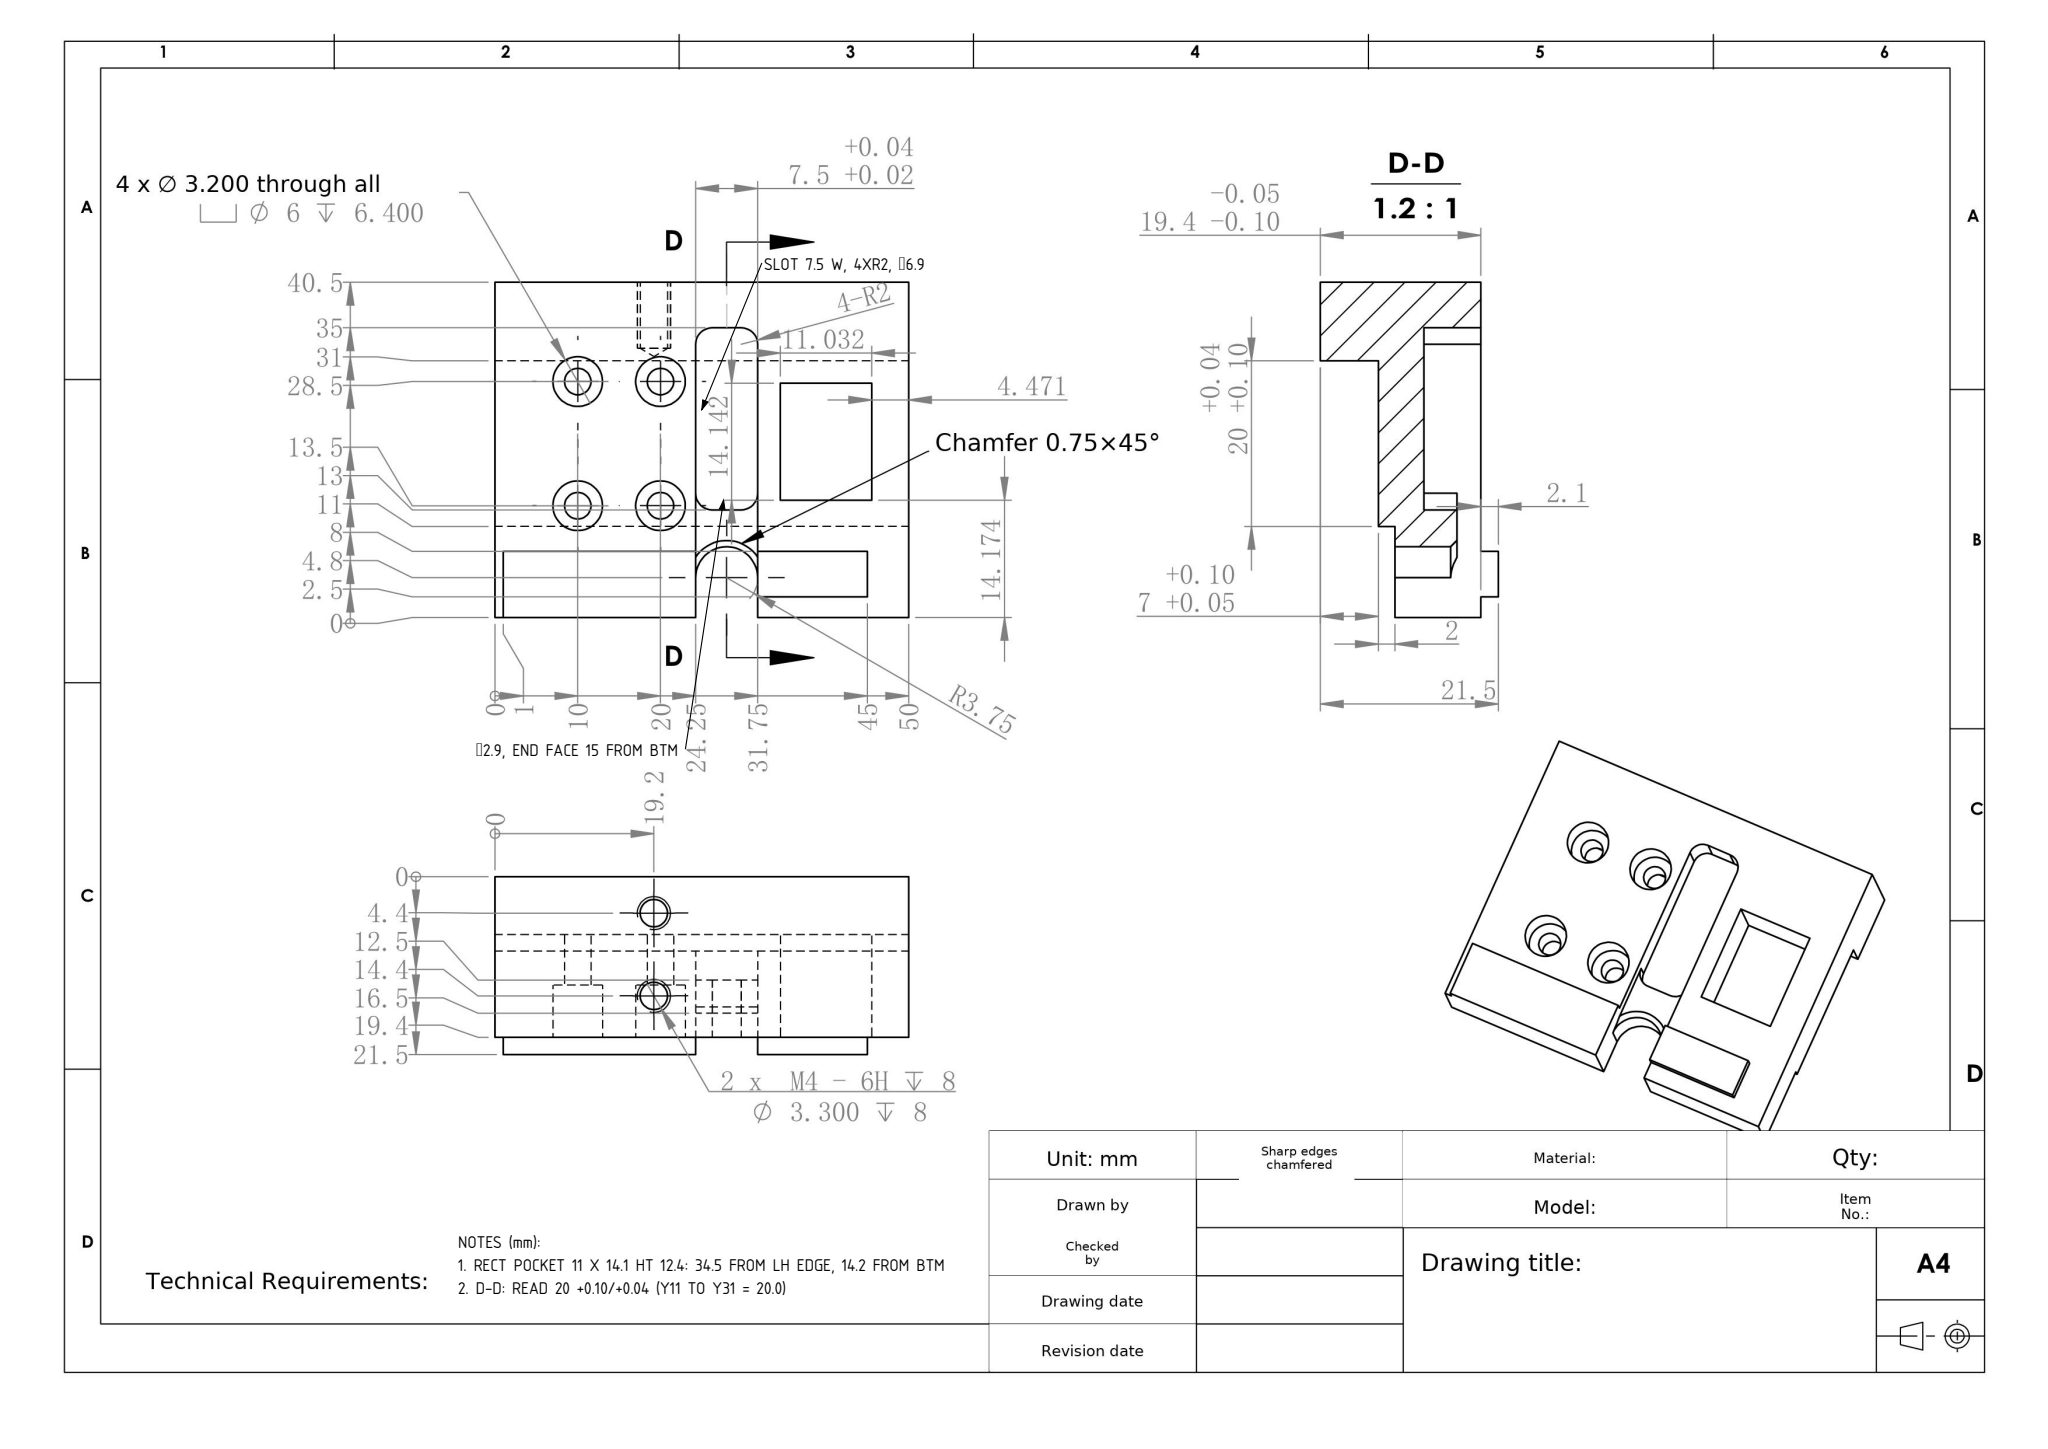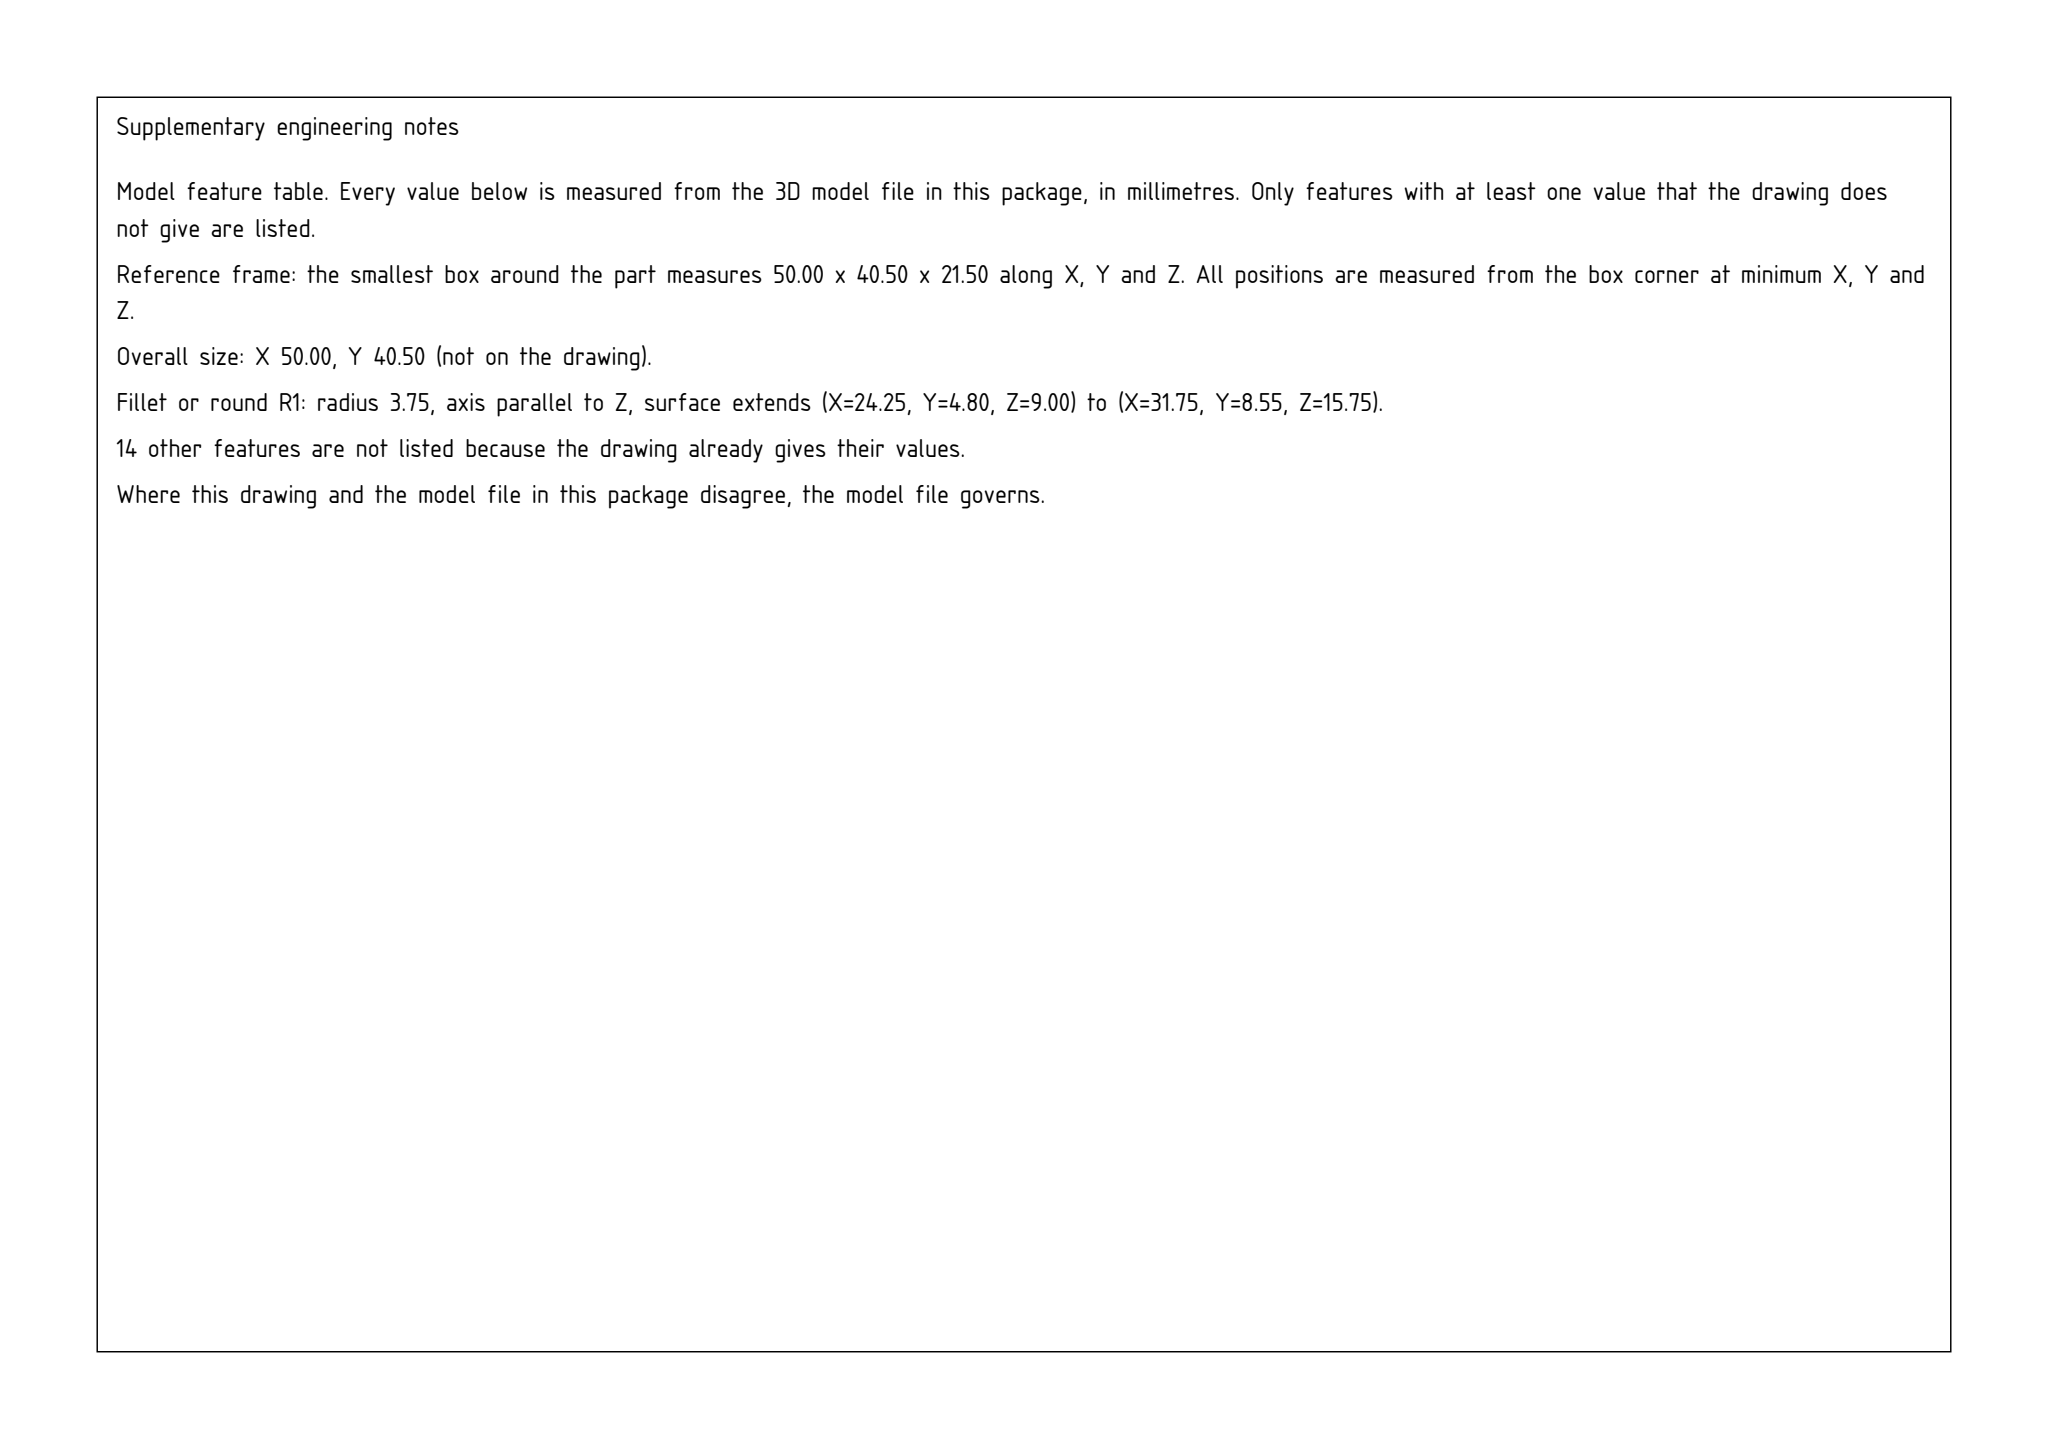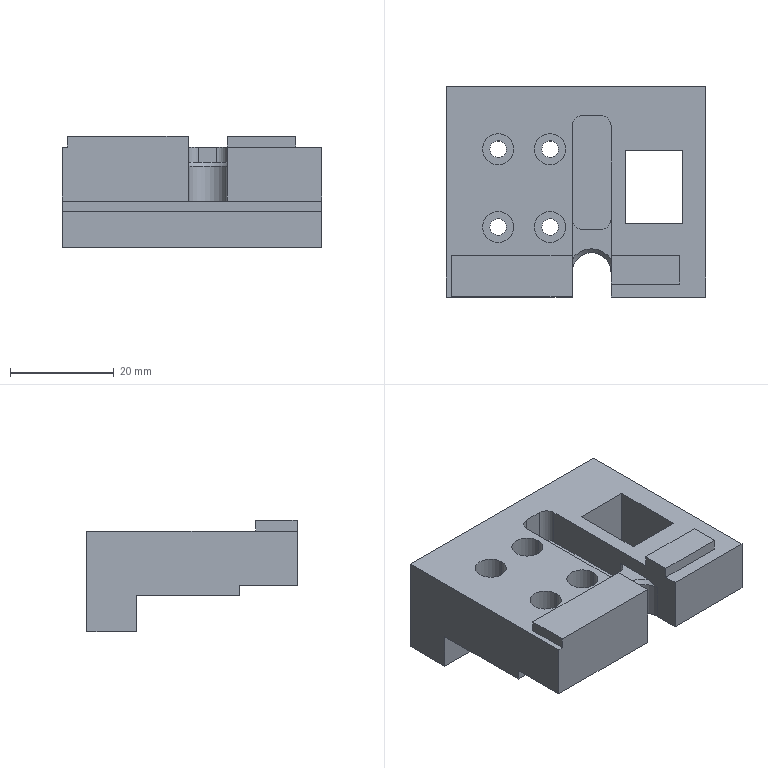Part | SolidWorks | mm | 1 solid | 62 faces | box 50 x 40.5 x 21.5 mm | volume 23052 mm3 | plane 32 | cylinder 25 | cone 5 | commonest cylinder face diameters 3.2 x8 6 x8 3.3 x4 4 x4 7.5 x1
Drawing notes:
ROUNDED SLOT (7.5 WIDE, 4-R2): OVERALL LENGTH 22.0, FROM Y 13.0 TO Y 35.0 FROM LOWER EDGE DATUM; DEPTH 6.9 FROM TOP FACE (floor at Z 12.5, top face Z 19.4); SLOT X 24.3 TO 31.8 FROM LEFT EDGE. | from the solid: axis_plane z=12.5 extent x[24.3,31.8] y[13.0,35.0]; planes y=13.0 and y=35.0 at x[26.3,29.8]; R2 arcs dia 4.0 at (26.3/29.8, 15.0/33.0)
RECT POCKET 11 X 14.1 HT 12.4: 34.5 FROM LH EDGE, 14.2 FROM BTM | from the solid: x-planes 34.5 & 45.5 (y 14.2-28.3, z 7.0-19.4); y-planes 14.2 & 28.3 (x 34.5-45.5); floor z=7.0, top face z=19.4 -> depth 12.4
STEP IN SLOT HT 2.9 FROM TOP: END FACE 15 FROM BTM EDGE | from the solid: z=16.5 face x 24.3-31.8, y 7.3-15.0; top z=19.4 -> 2.9 deep; step end at y=15 from y=0 edge
D-D: READ 20 +0.10/+0.04 (Y11 TO Y31 = 20.0) | from the solid: y-planes 11.0 and 31.0 across full x 0-50 -> 20.0 nominal; tolerance limits reversed on drawing